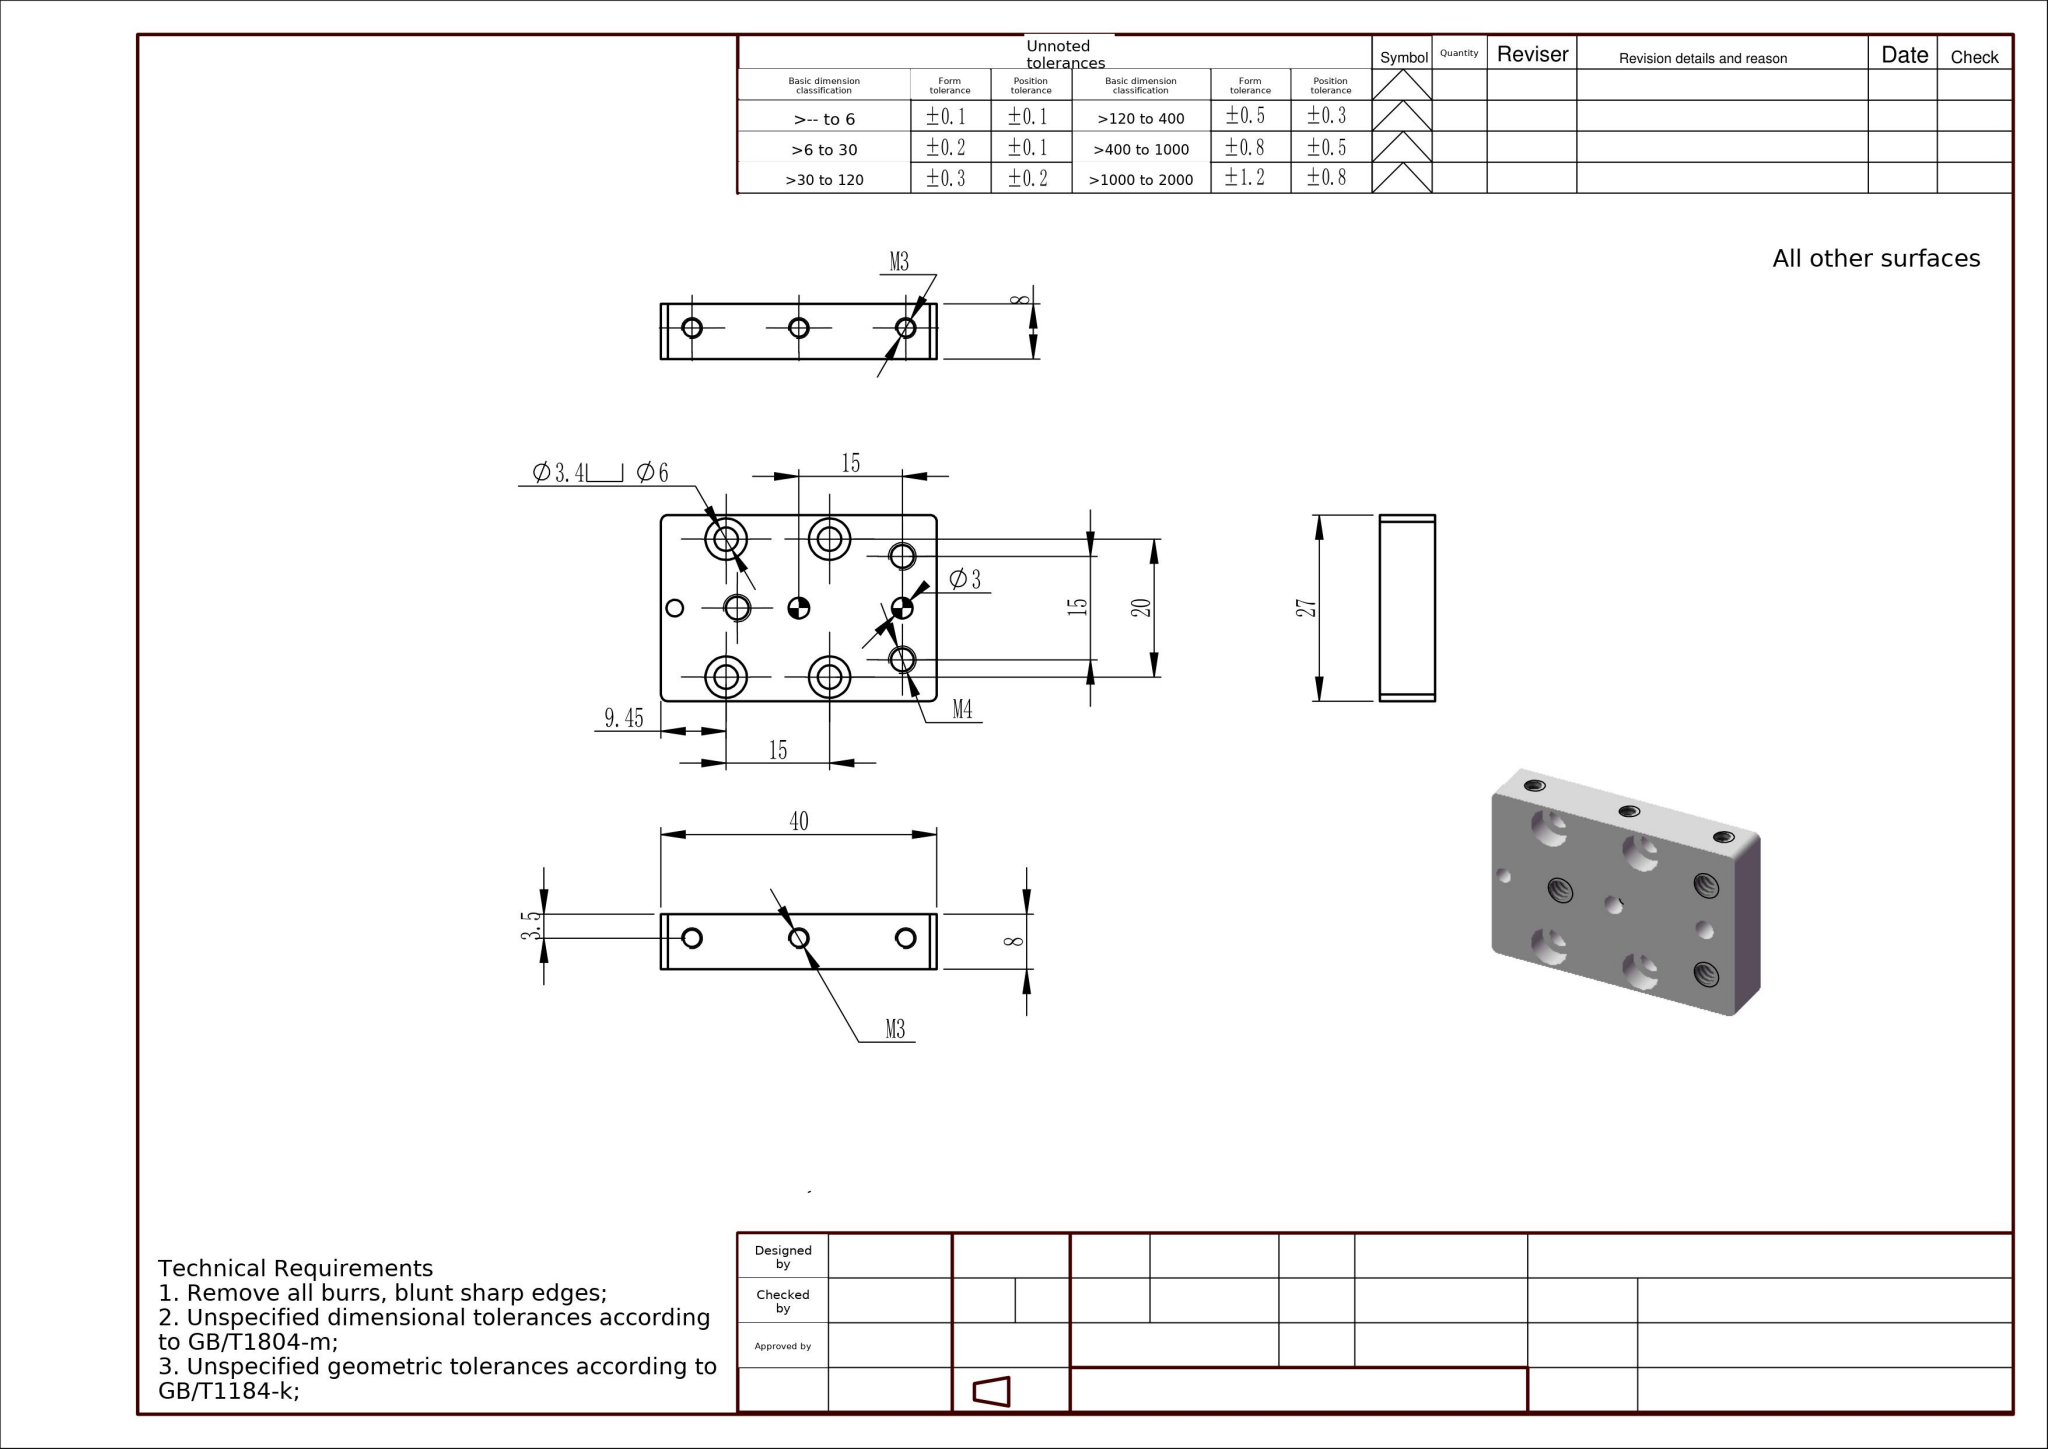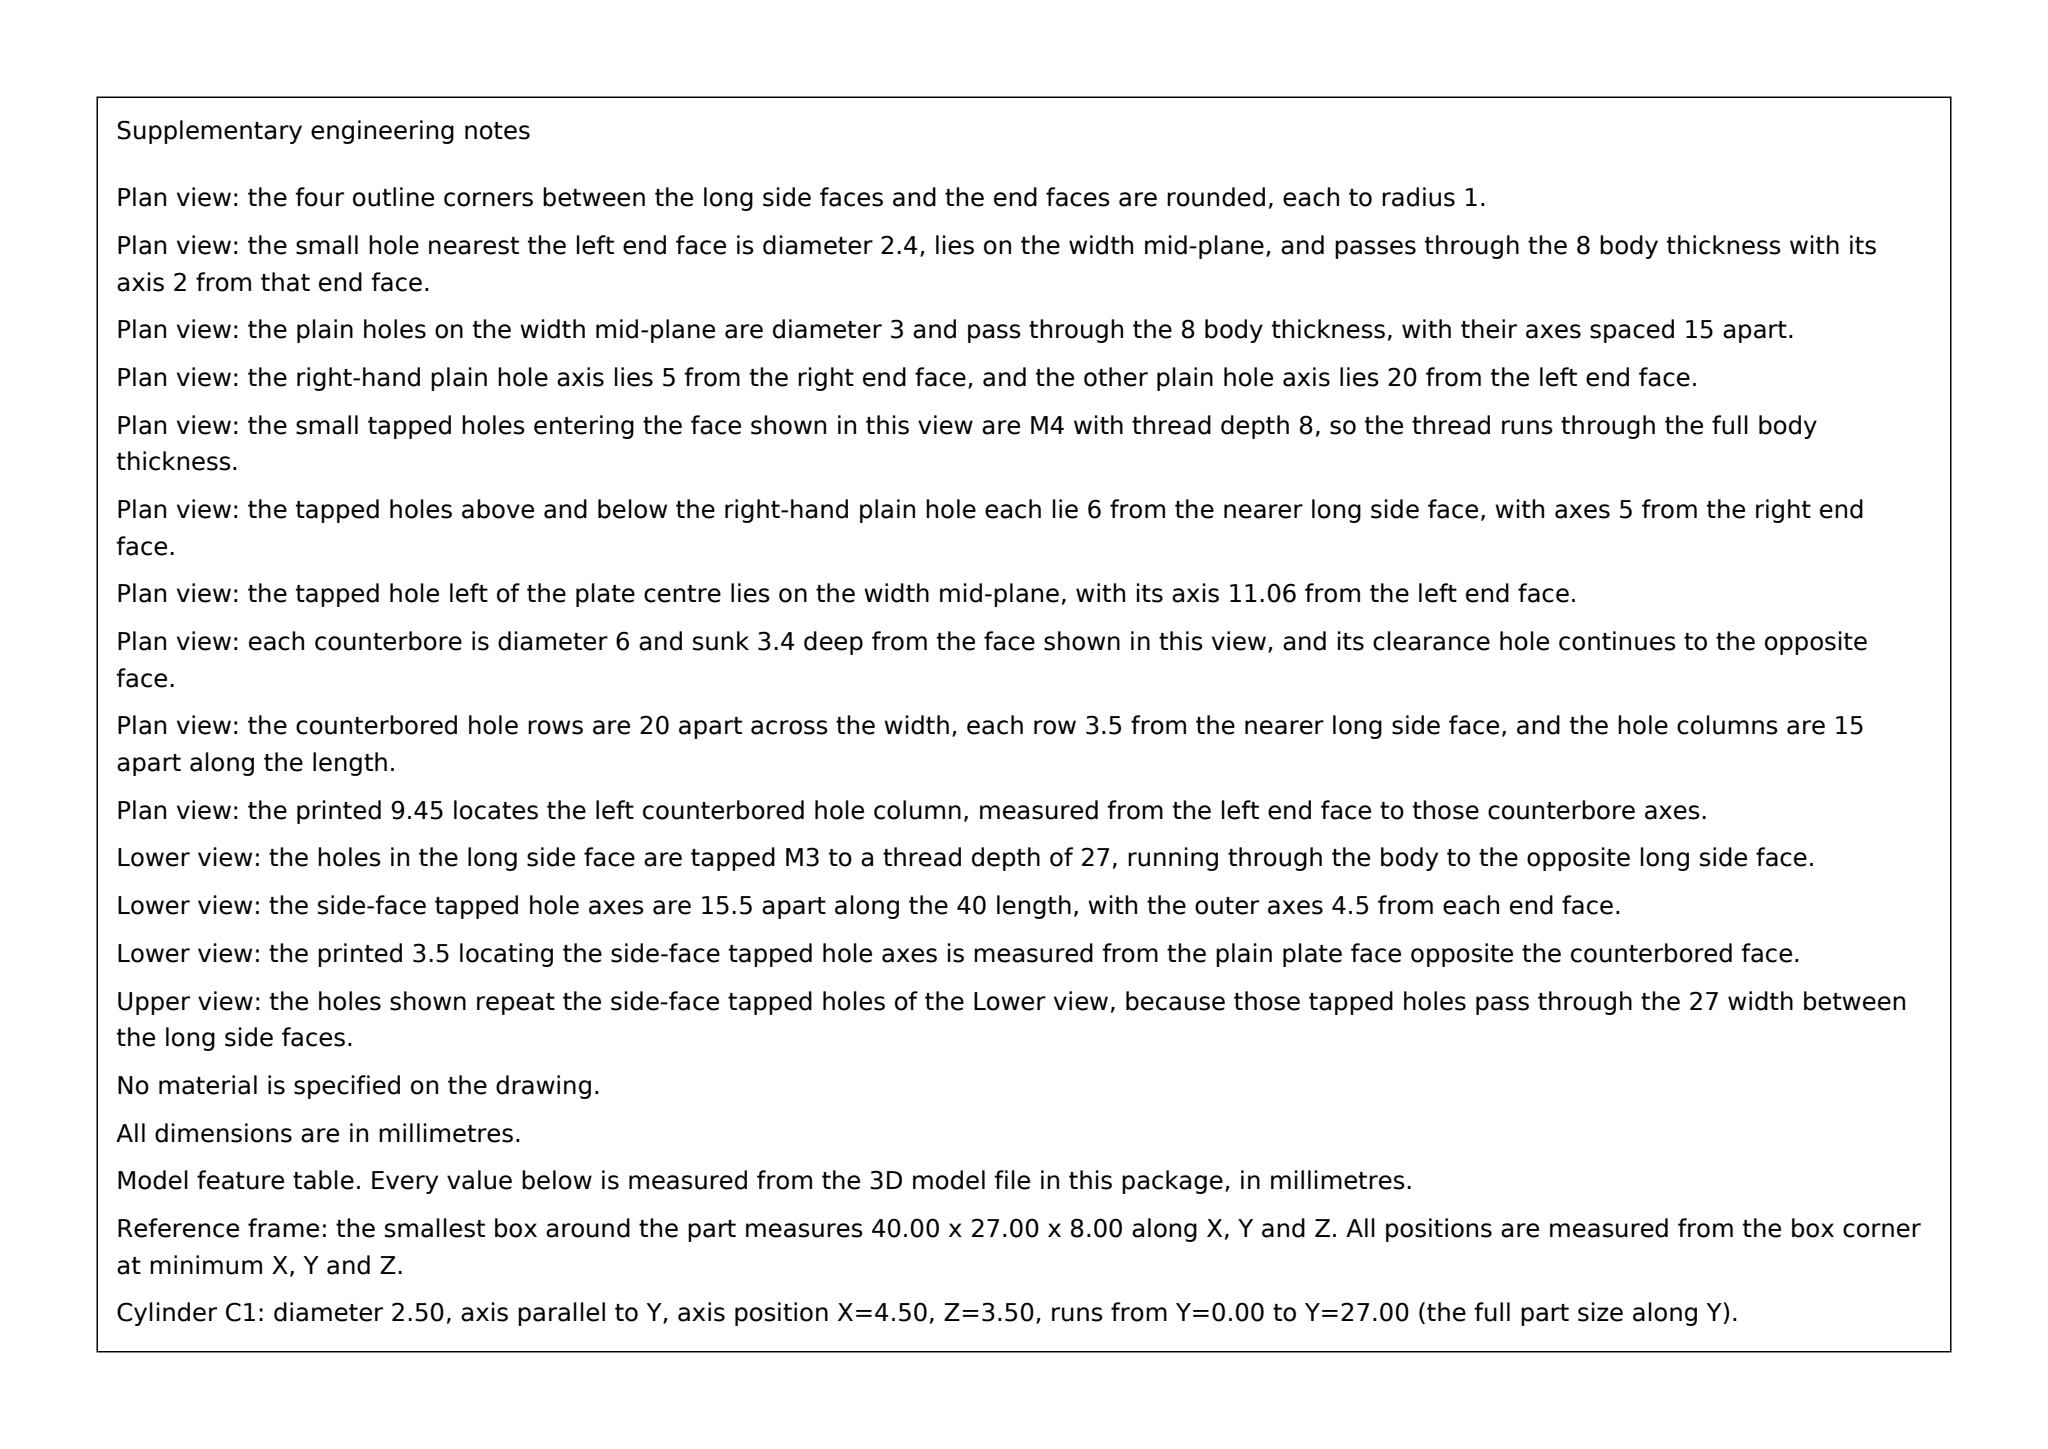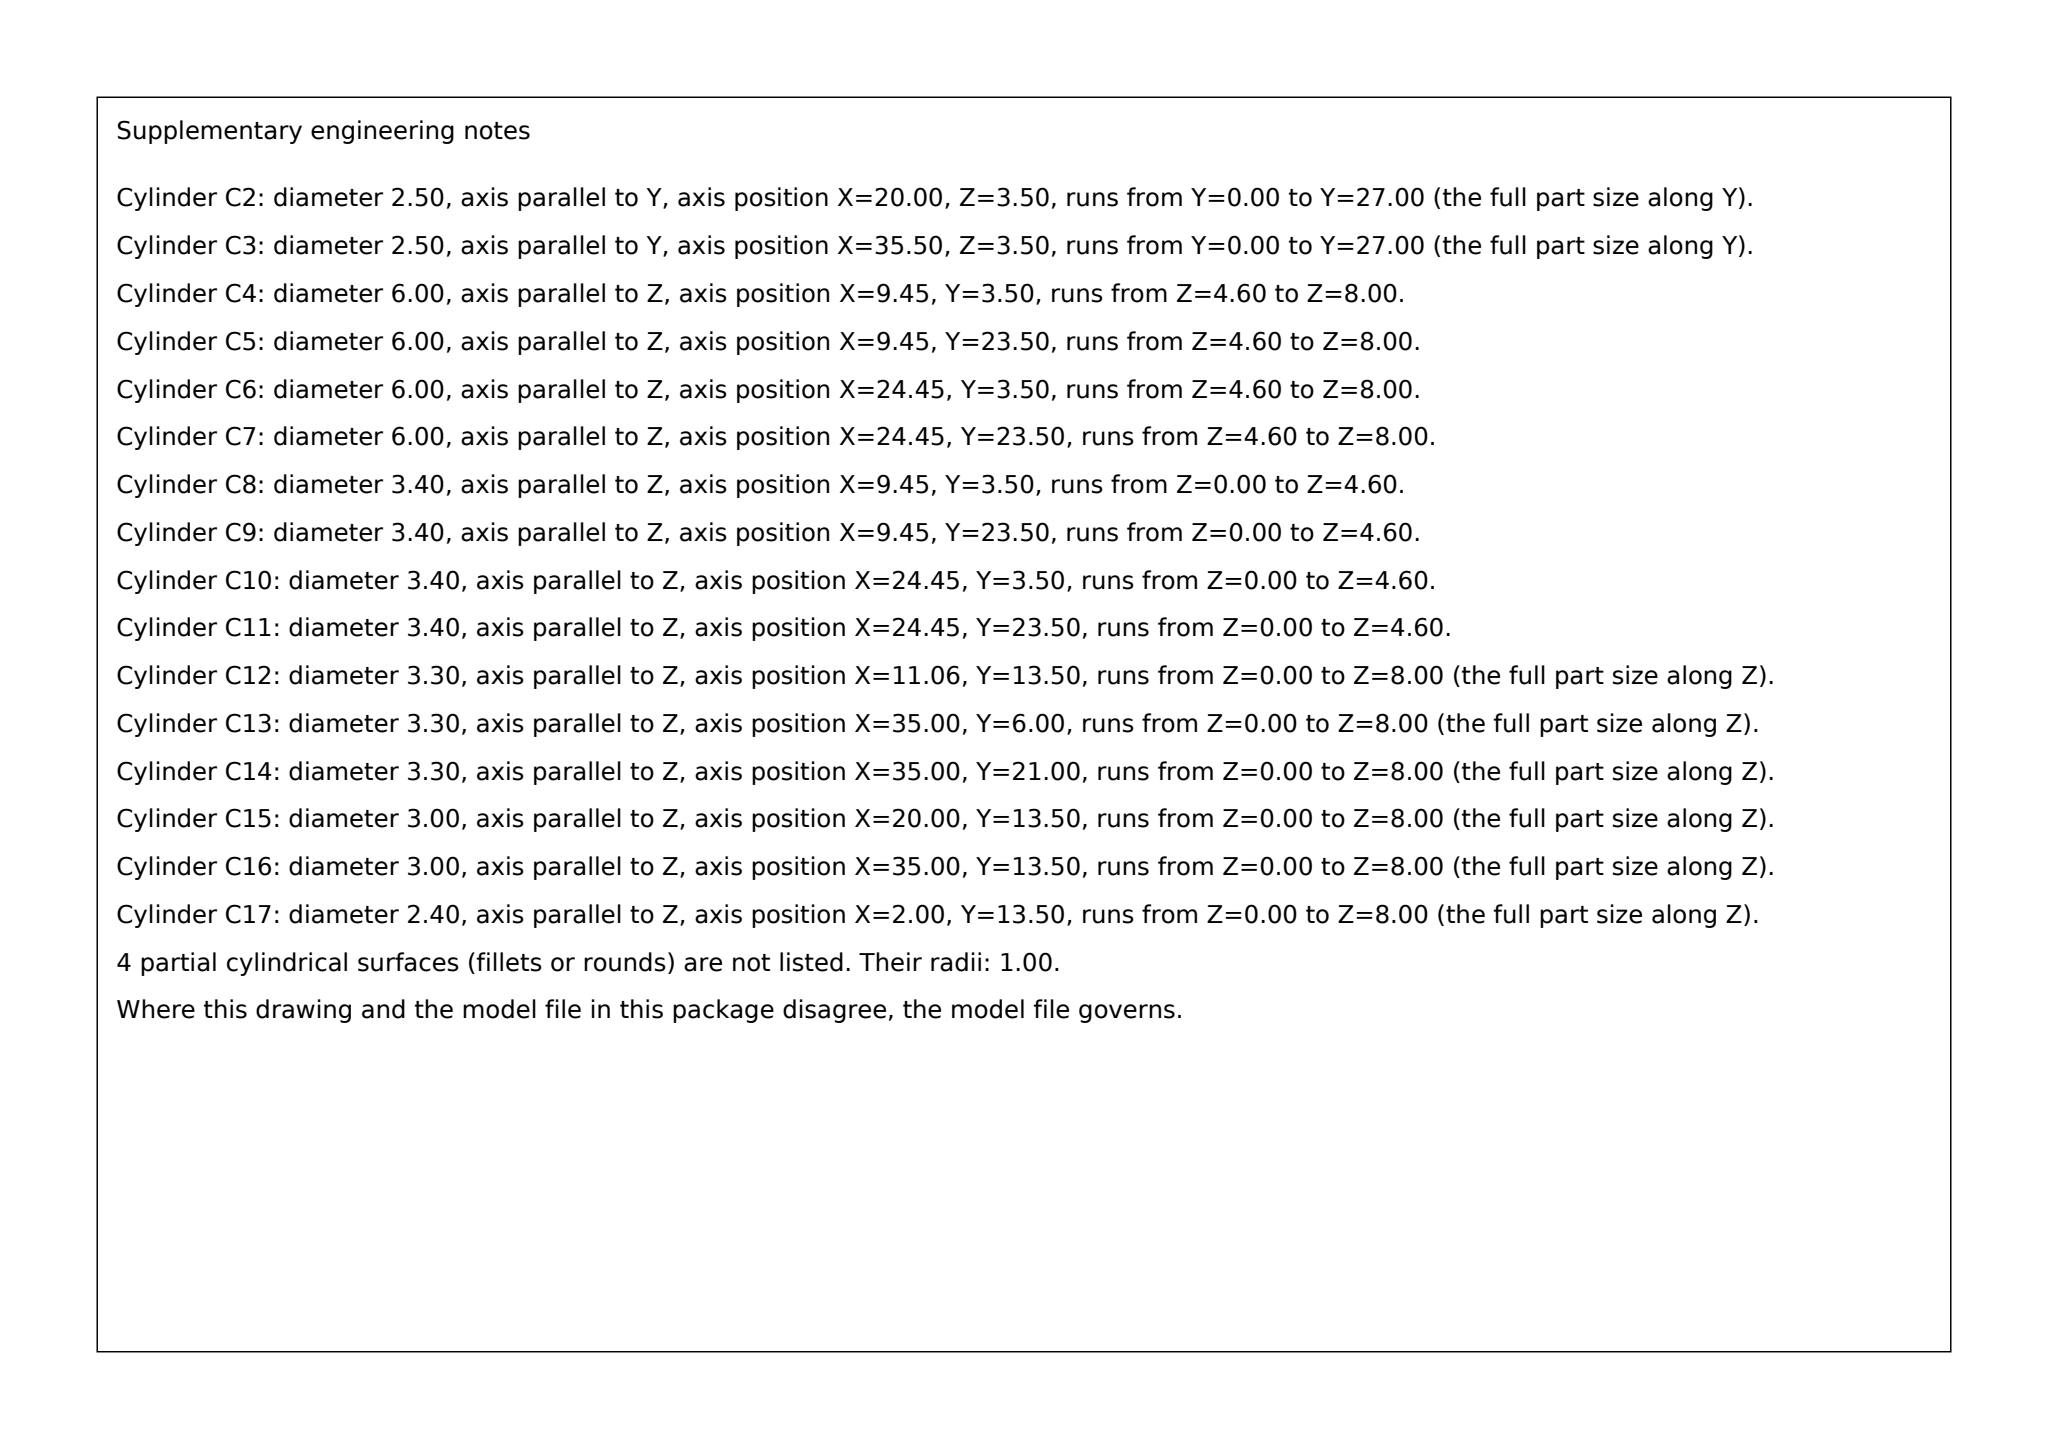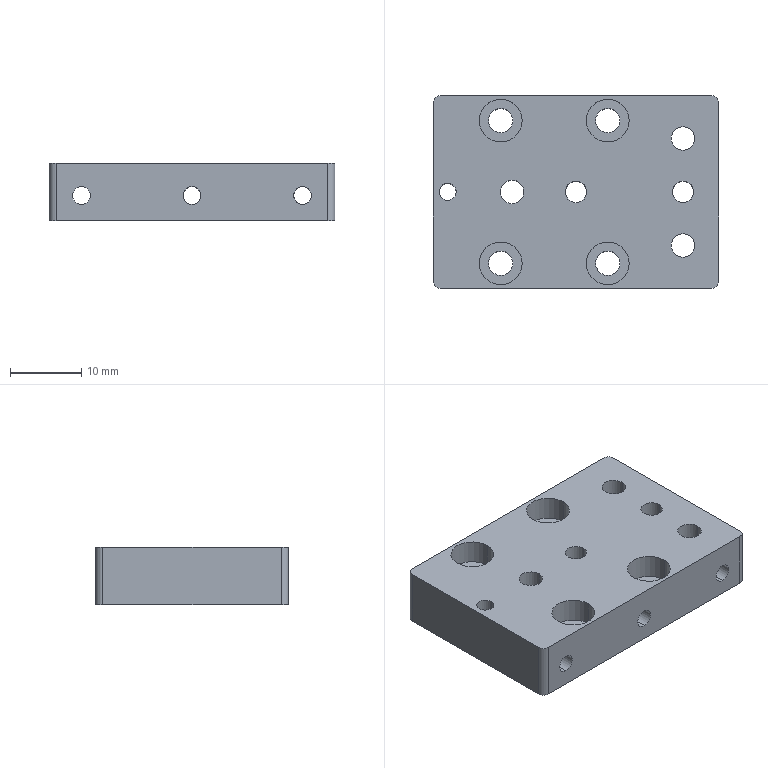Part | SolidWorks | mm | 1 solid | 53 faces | box 40 x 27 x 8 mm | volume 7382 mm3 | cylinder 43 | plane 10 | commonest cylinder face diameters 2.5 x11 6 x8 3.4 x8 3.3 x6 3 x4 2 x4 2.4 x2
Drawing notes:
M4 THRU, ON HORIZ CL, 11.06 FROM LH EDGE | from the solid: Ø3.3 cyl, axis z, pos (11.06,13.5), length 8 = full 8 thk (thru)
3X M4 THRU (Ø3.3 TAP DRILL) IN 40 X 27 FACE | from the solid: Ø3.3 cyls axis z at (11.06,13.5),(35,6),(35,21), each length 8 = thru
M3 THRU AT 4.5 & 35.5; CTR M3 (X20) DP 12.67 | from the solid: Ø2.5 cyls axis y, z=3.5: x=4.5 & 35.5 length 27 thru; x=20 length 12.67
build123d program:
from build123d import *

# Parameters (mm, degrees)
SKETCH1_W                                         = 40
SKETCH1_H                                         = 27
BOSS_EXTRUDE1_DEPTH                               = 8
HOLE_SIZE_ACCORDING_TO_HEXAGON_SOCKET_D           = 3.4
HOLE_SIZE_ACCORDING_TO_HEXAGON_SOCKET_CBORE_D     = 6
HOLE_SIZE_ACCORDING_TO_HEXAGON_SOCKET_CBORE_DEPTH = 3.4
M4_TAPPED_HOLE1_D                                 = 3.3
FILLET1_R                                         = 1
SIZE_MM_DOWEL_PIN_HOLE_1_D                        = 3
M3_TAPPED_HOLE3_D                                 = 2.5
F_2_4_2_4_DIAMETER_HOLE1_D                        = 2.4


with BuildPart() as part:
    # Sketch1 → Boss-Extrude1 (new body)
    with BuildSketch(Plane.XY):
        Rectangle(SKETCH1_W, SKETCH1_H)
    extrude(amount=BOSS_EXTRUDE1_DEPTH)

    # Hole Size _ According to_ Hexagon Socket (through all)
    with Locations(Plane(origin=(-10.55, -10, 8), x_dir=(1, 0, 0), z_dir=(0, 0, 1))):
        with Locations((0, 0), (0, 20), (15, 0), (15, 20)):
            CounterBoreHole(HOLE_SIZE_ACCORDING_TO_HEXAGON_SOCKET_D / 2, HOLE_SIZE_ACCORDING_TO_HEXAGON_SOCKET_CBORE_D / 2, HOLE_SIZE_ACCORDING_TO_HEXAGON_SOCKET_CBORE_DEPTH)

    # M4 Tapped Hole1 (through all)
    with Locations(Plane(origin=(15, 7.5, 8), x_dir=(1, 0, 0), z_dir=(0, 0, 1))):
        with Locations((0, 0), (0, -15), (-23.944, -7.5)):
            Hole(M4_TAPPED_HOLE1_D / 2)

    # Fillet1
    fillet1_edges = [part.edges().sort_by_distance(p)[0] for p in [
        (20, -13.5, 4),
        (-20, -13.5, 4),
        (-20, 13.5, 4),
        (20, 13.5, 4),
    ]]
    fillet(fillet1_edges, radius=FILLET1_R)

    # Size mm Dowel Pin Hole 1 (through all)
    with Locations(Plane.XY.offset(8)):
        with Locations((0, 0), (15, 0)):
            Hole(SIZE_MM_DOWEL_PIN_HOLE_1_D / 2)

    # M3 Tapped Hole3 (through all)
    with Locations(Plane(origin=(0, 13.5, 0), x_dir=(1, 0, 0), z_dir=(0, 1, 0))):
        with Locations((-15.5, -3.5), (0, -3.5), (15.5, -3.5)):
            Hole(M3_TAPPED_HOLE3_D / 2)

    # 2.4 _2.4_ Diameter Hole1 (through all)
    with Locations(Plane.XY.offset(8)):
        with Locations((-18, 0)):
            Hole(F_2_4_2_4_DIAMETER_HOLE1_D / 2)


solid = part.part